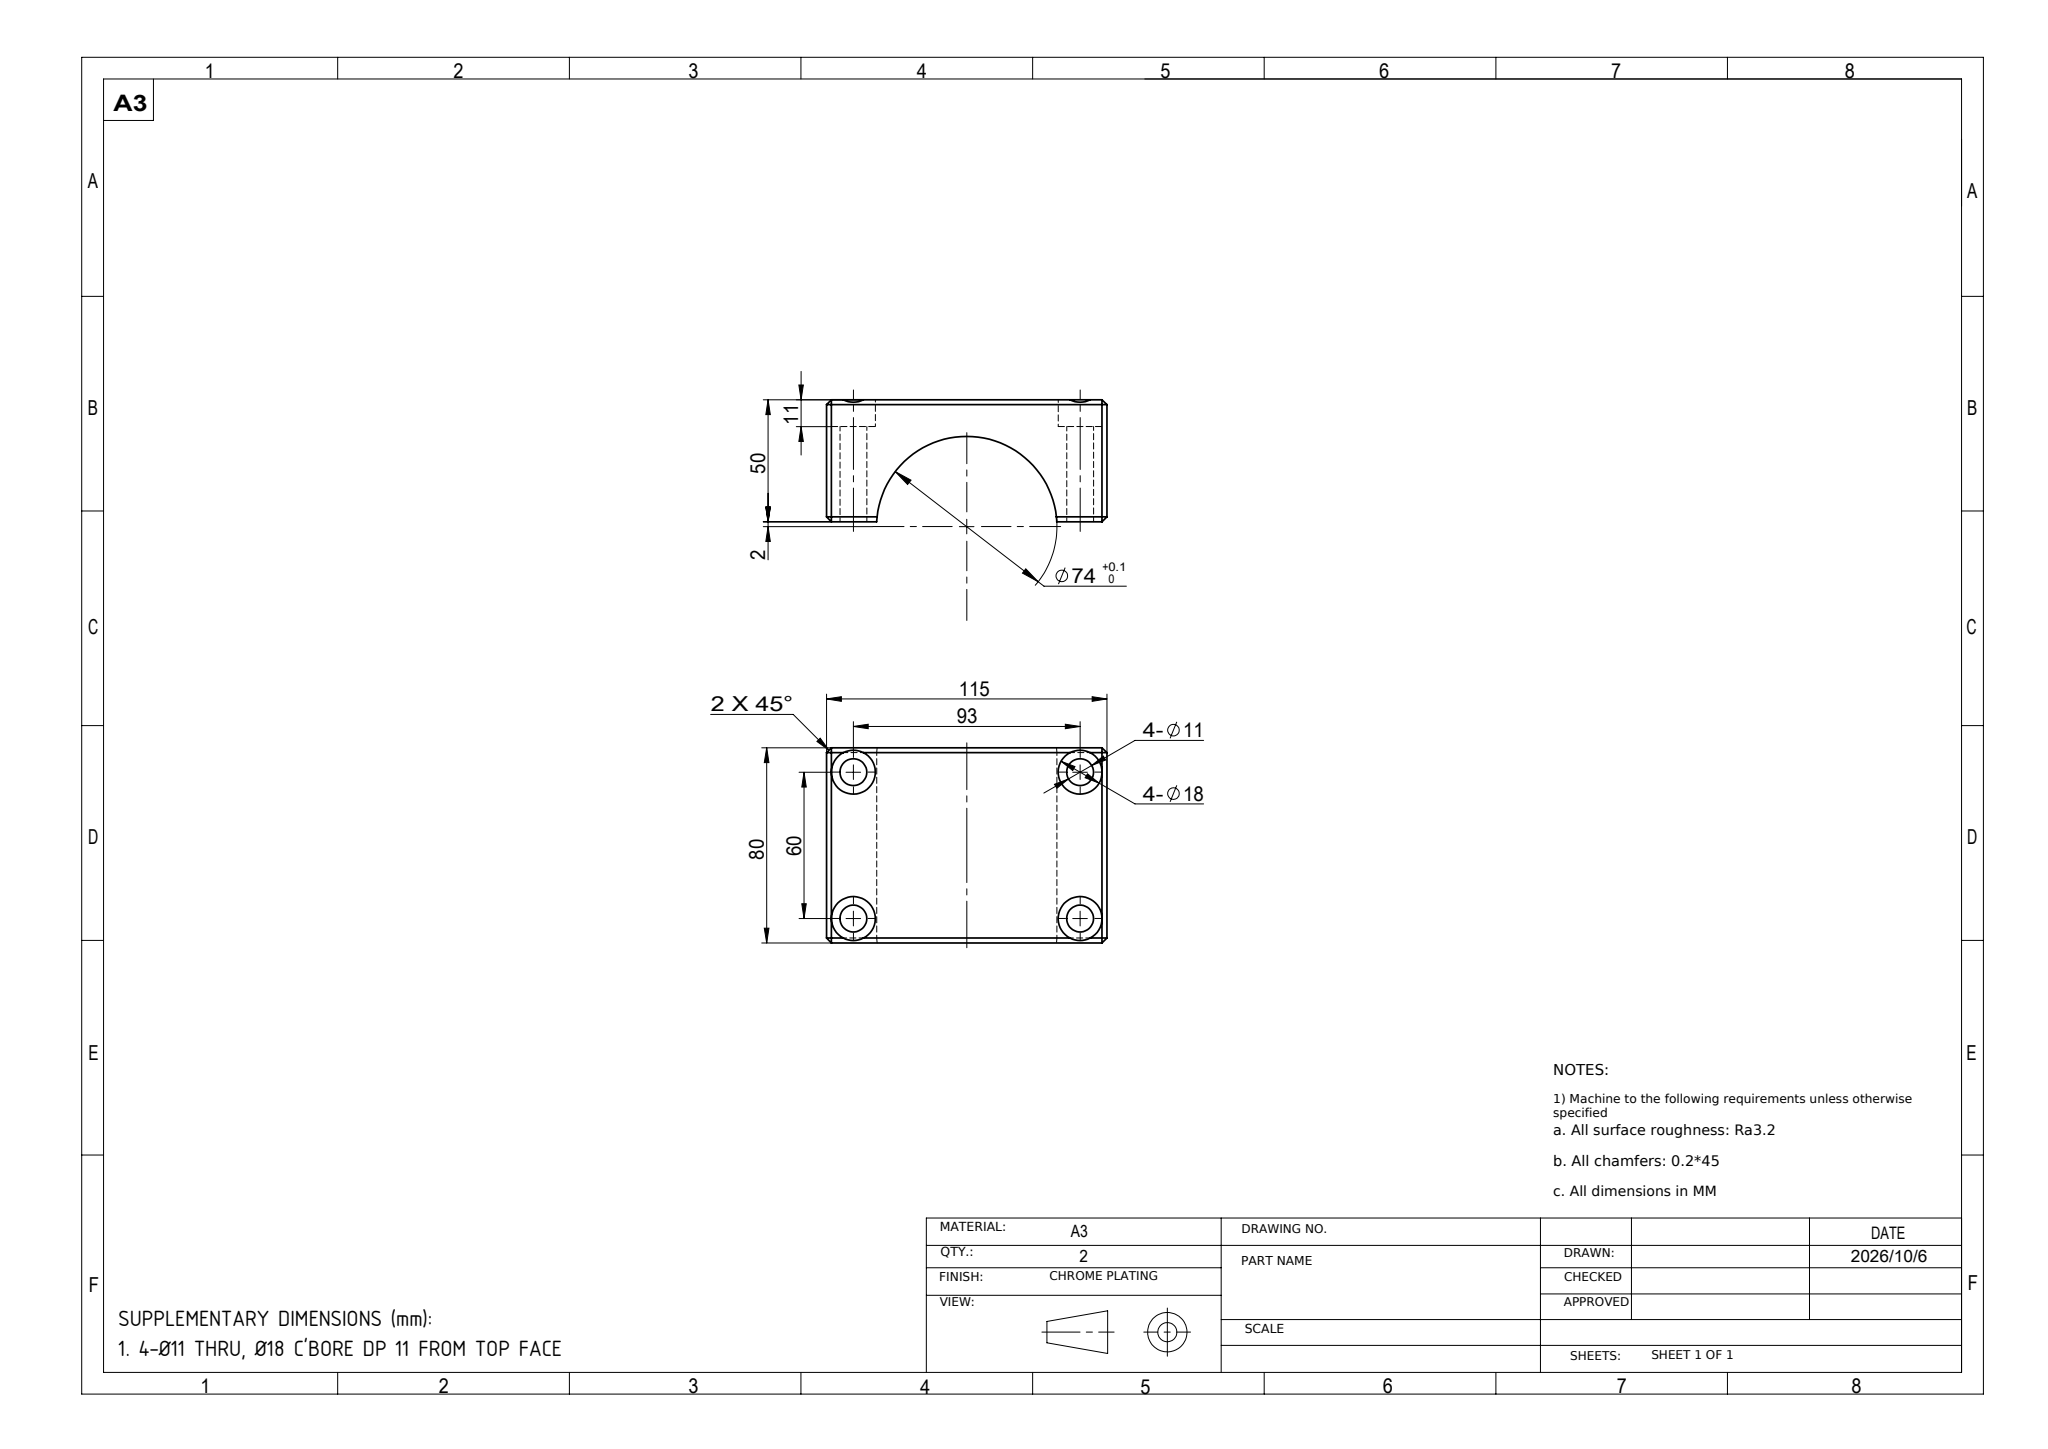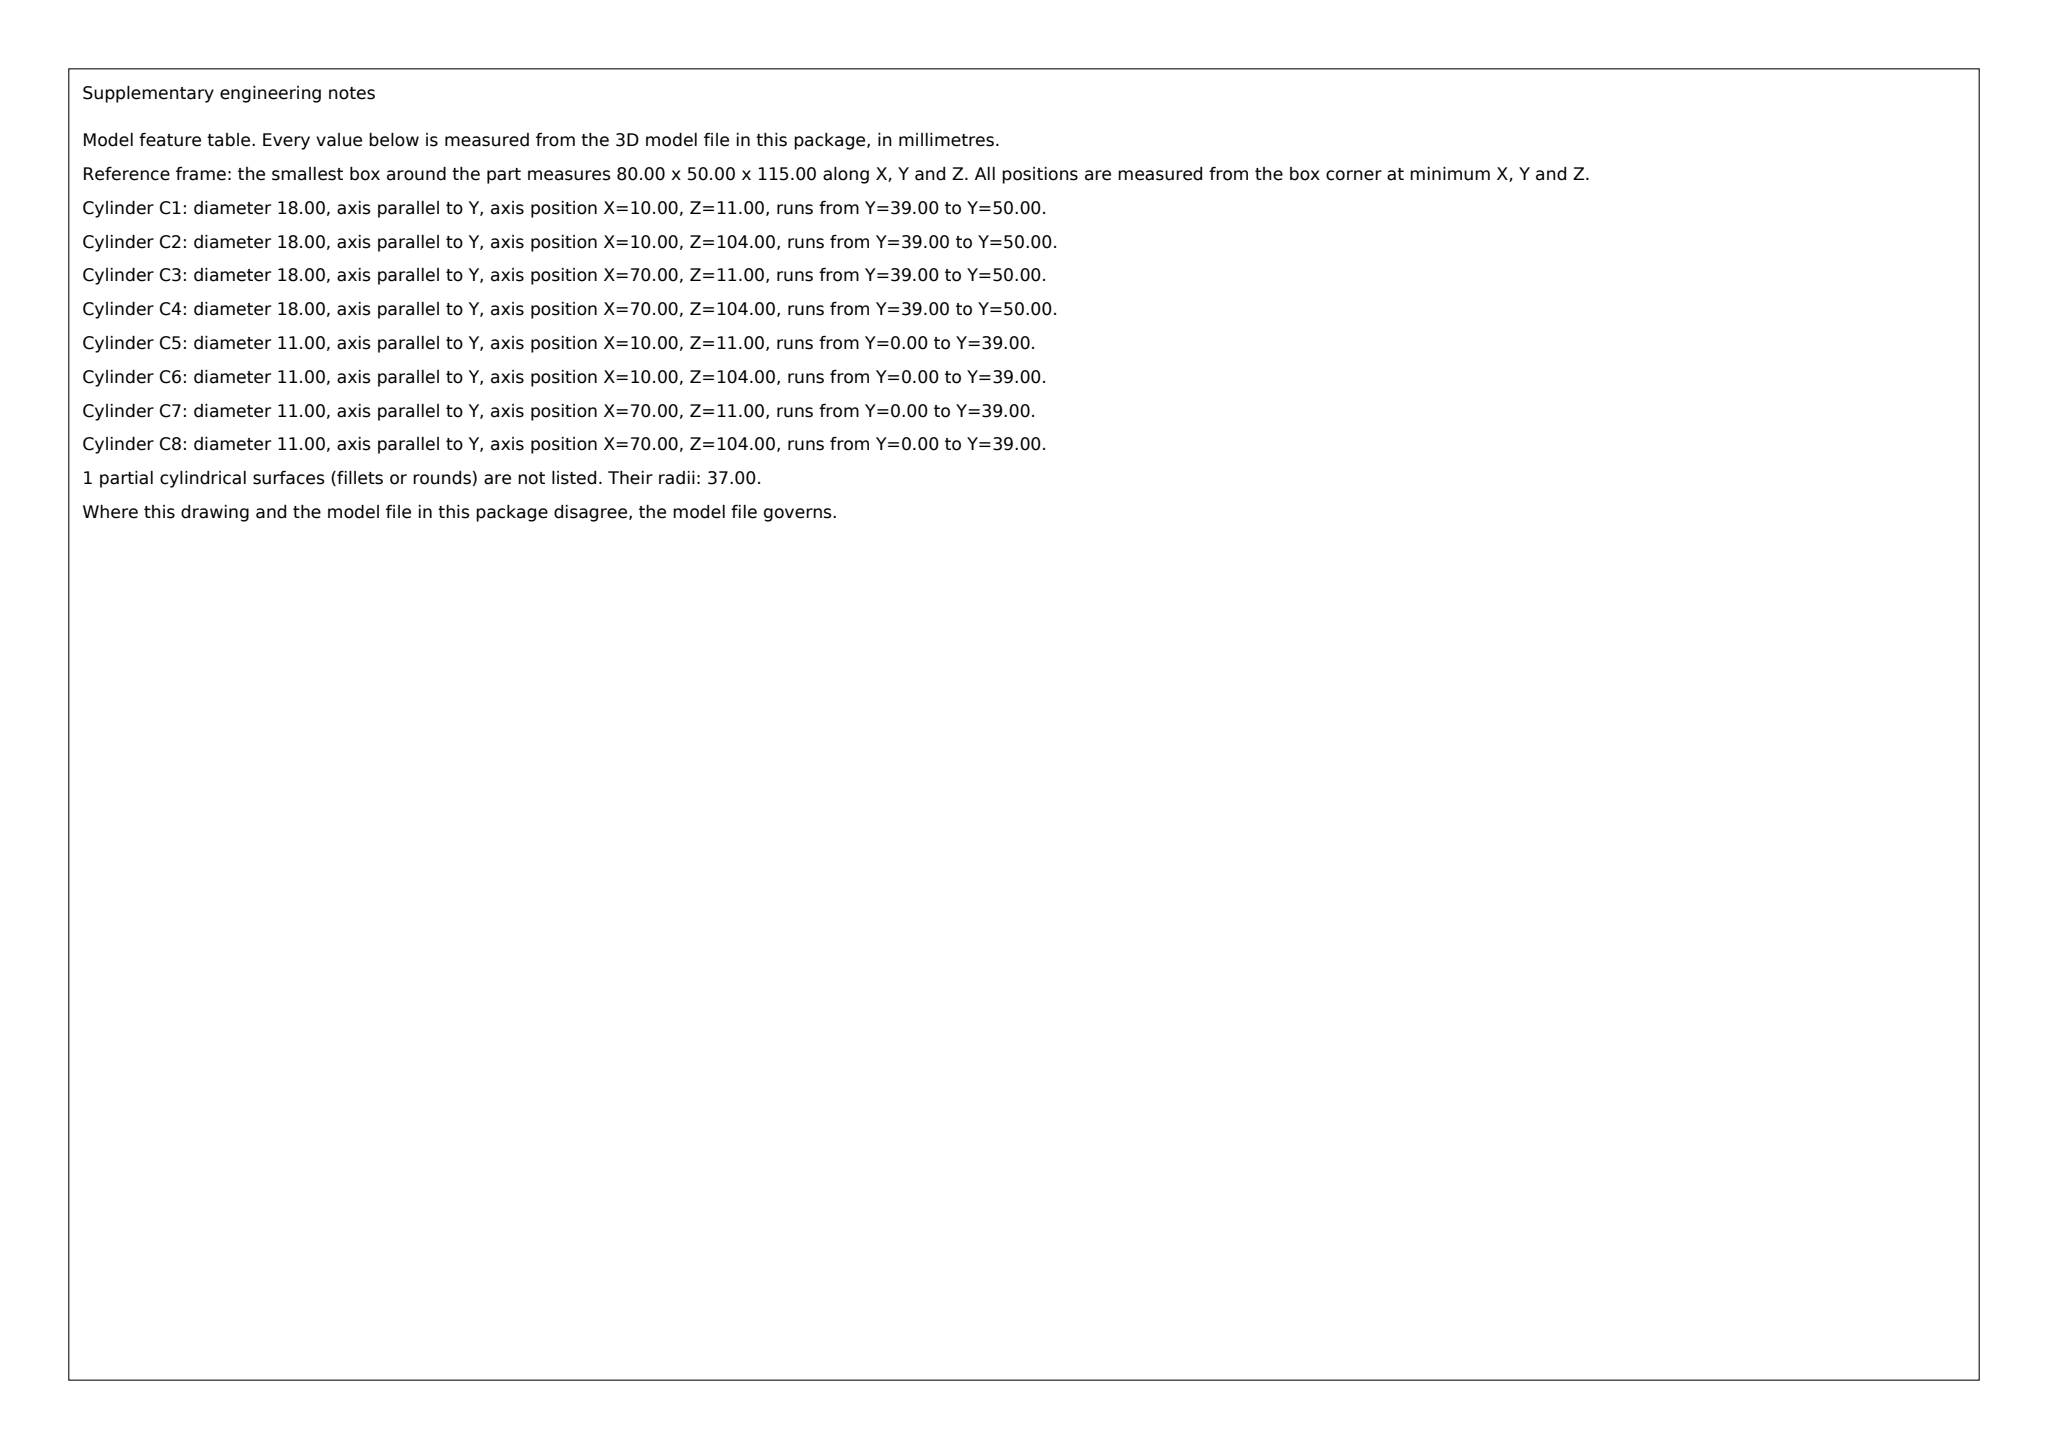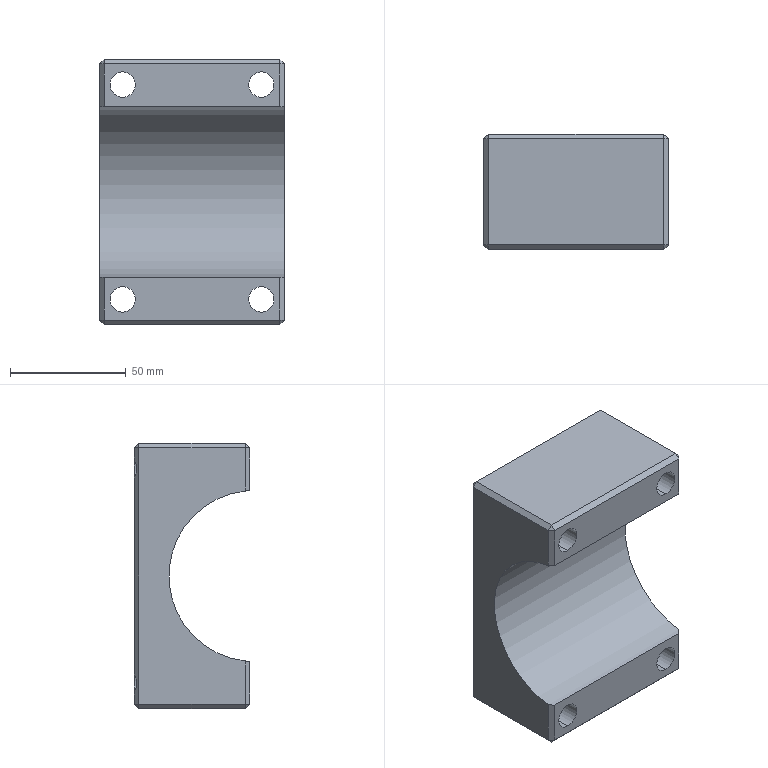Part | SolidWorks | mm | 1 solid | 54 faces | box 80 x 50 x 115 mm | volume 272166 mm3 | plane 37 | cylinder 17 | commonest cylinder face diameters 18 x8 11 x8 74 x1